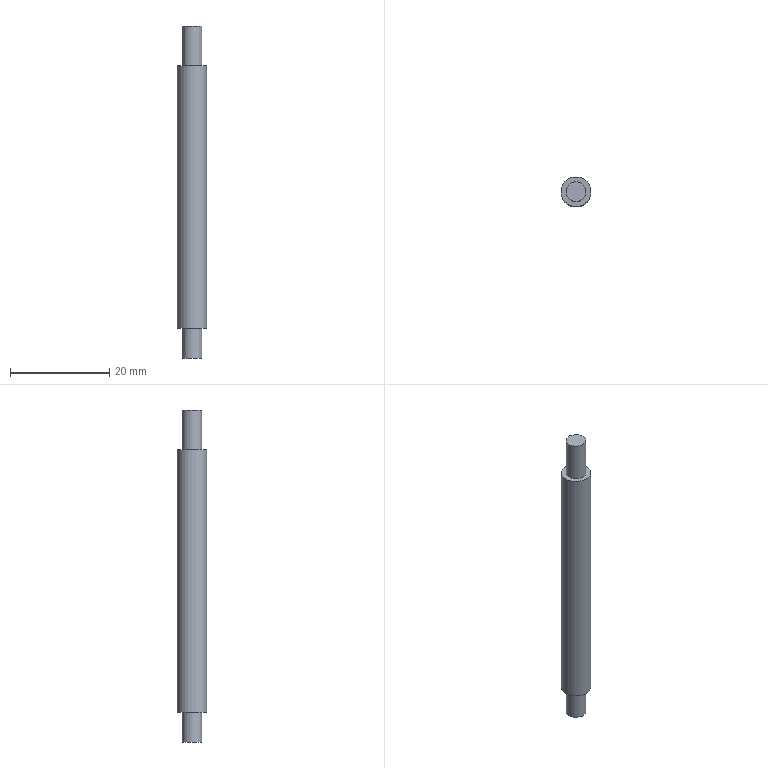Component | NX | CONN_ROD | 1 solid | 7 faces | box 6 x 6 x 67 mm | volume 1674 mm3 | plane 4 | cylinder 3 | commonest cylinder face diameters 4 x2 6 x1
STEP:
#1=CARTESIAN_POINT('',(0.,0.,0.));
#2=DIRECTION('',(0.,0.,1.));
#3=DIRECTION('',(1.,0.,0.));
#4=AXIS2_PLACEMENT_3D('',#1,#2,#3);
#5=CARTESIAN_POINT('',(2.,-10.,96.121));
#6=VERTEX_POINT('',#5);
#7=CARTESIAN_POINT('',(-0.,-10.,96.121));
#8=DIRECTION('',(0.,0.,1.));
#9=DIRECTION('',(1.,0.,0.));
#10=AXIS2_PLACEMENT_3D('',#7,#8,#9);
#11=CIRCLE('',#10,2.);
#12=CARTESIAN_POINT('',(-0.,-10.,96.121));
#13=DIRECTION('',(0.,0.,-1.));
#14=DIRECTION('',(-1.,0.,0.));
#15=AXIS2_PLACEMENT_3D('',#12,#13,#14);
#16=PLANE('',#15);
#17=CARTESIAN_POINT('',(-2.,0.));
#18=CARTESIAN_POINT('',(-2.,3.464));
#19=CARTESIAN_POINT('',(1.,1.732));
#20=CARTESIAN_POINT('',(4.,0.));
#21=CARTESIAN_POINT('',(1.,-1.732));
#22=CARTESIAN_POINT('',(-2.,-3.464));
#23=CARTESIAN_POINT('',(-2.,0.));
#24=(BOUNDED_CURVE()B_SPLINE_CURVE(2,(#17,#18,#19,#20,#21,#22,#23),.UNSPECIFIED.,.T.,.F.)B_SPLINE_CURVE_WITH_KNOTS((1,2,2,2,2,1),(-2.094,0.,2.094,4.189,6.283,8.378),.UNSPECIFIED.)CURVE()GEOMETRIC_REPRESENTATION_ITEM()RATIONAL_B_SPLINE_CURVE((1.,0.5,1.,0.5,1.,0.5,1.))REPRESENTATION_ITEM(''));
#25=(GEOMETRIC_REPRESENTATION_CONTEXT(2)PARAMETRIC_REPRESENTATION_CONTEXT()REPRESENTATION_CONTEXT('',''));
#26=DEFINITIONAL_REPRESENTATION('',(#24),#25);
#27=PCURVE('',#16,#26);
#28=CARTESIAN_POINT('',(-0.,-10.,96.121));
#29=DIRECTION('',(0.,0.,1.));
#30=DIRECTION('',(1.,0.,0.));
#31=AXIS2_PLACEMENT_3D('',#28,#29,#30);
#32=CYLINDRICAL_SURFACE('',#31,2.);
#33=CARTESIAN_POINT('',(0.,0.));
#34=DIRECTION('',(1.,0.));
#35=VECTOR('',#34,1.);
#36=LINE('',#33,#35);
#37=(GEOMETRIC_REPRESENTATION_CONTEXT(2)PARAMETRIC_REPRESENTATION_CONTEXT()REPRESENTATION_CONTEXT('',''));
#38=DEFINITIONAL_REPRESENTATION('',(#36),#37);
#39=PCURVE('',#32,#38);
#40=SURFACE_CURVE('',#11,(#27,#39),.PCURVE_S1.);
#41=EDGE_CURVE('',#6,#6,#40,.T.);
#42=ORIENTED_EDGE('',*,*,#41,.F.);
#43=EDGE_LOOP('',(#42));
#44=FACE_BOUND('',#43,.T.);
#45=ADVANCED_FACE('',(#44),#16,.T.);
#46=CARTESIAN_POINT('',(2.,-10.,102.121));
#47=VERTEX_POINT('',#46);
#48=CARTESIAN_POINT('',(-0.,-10.,102.121));
#49=DIRECTION('',(0.,0.,-1.));
#50=DIRECTION('',(1.,0.,0.));
#51=AXIS2_PLACEMENT_3D('',#48,#49,#50);
#52=CIRCLE('',#51,2.);
#53=CARTESIAN_POINT('',(6.283,6.));
#54=DIRECTION('',(-1.,0.));
#55=VECTOR('',#54,1.);
#56=LINE('',#53,#55);
#57=(GEOMETRIC_REPRESENTATION_CONTEXT(2)PARAMETRIC_REPRESENTATION_CONTEXT()REPRESENTATION_CONTEXT('',''));
#58=DEFINITIONAL_REPRESENTATION('',(#56),#57);
#59=PCURVE('',#32,#58);
#60=CARTESIAN_POINT('',(-0.,-10.,102.121));
#61=DIRECTION('',(0.,0.,-1.));
#62=DIRECTION('',(-1.,0.,0.));
#63=AXIS2_PLACEMENT_3D('',#60,#61,#62);
#64=PLANE('',#63);
#65=CARTESIAN_POINT('',(0.,0.));
#66=DIRECTION('',(-1.,0.));
#67=AXIS2_PLACEMENT_2D('',#65,#66);
#68=CIRCLE('',#67,2.);
#69=(GEOMETRIC_REPRESENTATION_CONTEXT(2)PARAMETRIC_REPRESENTATION_CONTEXT()REPRESENTATION_CONTEXT('',''));
#70=DEFINITIONAL_REPRESENTATION('',(#68),#69);
#71=PCURVE('',#64,#70);
#72=SURFACE_CURVE('',#52,(#59,#71),.PCURVE_S1.);
#73=EDGE_CURVE('',#47,#47,#72,.T.);
#74=ORIENTED_EDGE('',*,*,#73,.T.);
#75=CARTESIAN_POINT('',(2.,-10.,96.121));
#76=CARTESIAN_POINT('',(2.,-10.,102.121));
#77=B_SPLINE_CURVE_WITH_KNOTS('',1,(#75,#76),.UNSPECIFIED.,.F.,.F.,(2,2),(0.,6.),.PIECEWISE_BEZIER_KNOTS.);
#78=CARTESIAN_POINT('',(0.,0.));
#79=DIRECTION('',(0.,1.));
#80=VECTOR('',#79,1.);
#81=LINE('',#78,#80);
#82=(GEOMETRIC_REPRESENTATION_CONTEXT(2)PARAMETRIC_REPRESENTATION_CONTEXT()REPRESENTATION_CONTEXT('',''));
#83=DEFINITIONAL_REPRESENTATION('',(#81),#82);
#84=PCURVE('',#32,#83);
#85=CARTESIAN_POINT('',(6.283,0.));
#86=DIRECTION('',(0.,1.));
#87=VECTOR('',#86,1.);
#88=LINE('',#85,#87);
#89=(GEOMETRIC_REPRESENTATION_CONTEXT(2)PARAMETRIC_REPRESENTATION_CONTEXT()REPRESENTATION_CONTEXT('',''));
#90=DEFINITIONAL_REPRESENTATION('',(#88),#89);
#91=PCURVE('',#32,#90);
#92=SEAM_CURVE('',#77,(#84,#91),.PCURVE_S1.);
#93=EDGE_CURVE('',#6,#47,#92,.T.);
#94=ORIENTED_EDGE('',*,*,#93,.F.);
#95=ORIENTED_EDGE('',*,*,#41,.T.);
#96=ORIENTED_EDGE('',*,*,#93,.T.);
#97=EDGE_LOOP('',(#74,#94,#95,#96));
#98=FACE_BOUND('',#97,.T.);
#99=ADVANCED_FACE('',(#98),#32,.T.);
#100=CARTESIAN_POINT('',(2.,-10.,155.121));
#101=VERTEX_POINT('',#100);
#102=CARTESIAN_POINT('',(-0.,-10.,155.121));
#103=DIRECTION('',(0.,0.,1.));
#104=DIRECTION('',(1.,0.,0.));
#105=AXIS2_PLACEMENT_3D('',#102,#103,#104);
#106=CIRCLE('',#105,2.);
#107=CARTESIAN_POINT('',(-0.,-10.,155.121));
#108=DIRECTION('',(0.,0.,1.));
#109=DIRECTION('',(1.,0.,0.));
#110=AXIS2_PLACEMENT_3D('',#107,#108,#109);
#111=PLANE('',#110);
#112=CARTESIAN_POINT('',(0.,0.));
#113=DIRECTION('',(1.,0.));
#114=AXIS2_PLACEMENT_2D('',#112,#113);
#115=CIRCLE('',#114,2.);
#116=(GEOMETRIC_REPRESENTATION_CONTEXT(2)PARAMETRIC_REPRESENTATION_CONTEXT()REPRESENTATION_CONTEXT('',''));
#117=DEFINITIONAL_REPRESENTATION('',(#115),#116);
#118=PCURVE('',#111,#117);
#119=CARTESIAN_POINT('',(-0.,-10.,155.121));
#120=DIRECTION('',(0.,0.,1.));
#121=DIRECTION('',(1.,0.,0.));
#122=AXIS2_PLACEMENT_3D('',#119,#120,#121);
#123=CYLINDRICAL_SURFACE('',#122,2.);
#124=CARTESIAN_POINT('',(0.,0.));
#125=DIRECTION('',(1.,0.));
#126=VECTOR('',#125,1.);
#127=LINE('',#124,#126);
#128=(GEOMETRIC_REPRESENTATION_CONTEXT(2)PARAMETRIC_REPRESENTATION_CONTEXT()REPRESENTATION_CONTEXT('',''));
#129=DEFINITIONAL_REPRESENTATION('',(#127),#128);
#130=PCURVE('',#123,#129);
#131=SURFACE_CURVE('',#106,(#118,#130),.PCURVE_S1.);
#132=EDGE_CURVE('',#101,#101,#131,.T.);
#133=ORIENTED_EDGE('',*,*,#132,.F.);
#134=EDGE_LOOP('',(#133));
#135=FACE_BOUND('',#134,.T.);
#136=CARTESIAN_POINT('',(3.,-10.,155.121));
#137=VERTEX_POINT('',#136);
#138=CARTESIAN_POINT('',(-0.,-10.,155.121));
#139=DIRECTION('',(0.,0.,1.));
#140=DIRECTION('',(1.,0.,0.));
#141=AXIS2_PLACEMENT_3D('',#138,#139,#140);
#142=CIRCLE('',#141,3.);
#143=CARTESIAN_POINT('',(0.,0.));
#144=DIRECTION('',(1.,0.));
#145=AXIS2_PLACEMENT_2D('',#143,#144);
#146=CIRCLE('',#145,3.);
#147=(GEOMETRIC_REPRESENTATION_CONTEXT(2)PARAMETRIC_REPRESENTATION_CONTEXT()REPRESENTATION_CONTEXT('',''));
#148=DEFINITIONAL_REPRESENTATION('',(#146),#147);
#149=PCURVE('',#111,#148);
#150=CARTESIAN_POINT('',(-0.,-10.,102.121));
#151=DIRECTION('',(0.,0.,1.));
#152=DIRECTION('',(1.,0.,0.));
#153=AXIS2_PLACEMENT_3D('',#150,#151,#152);
#154=CYLINDRICAL_SURFACE('',#153,3.);
#155=CARTESIAN_POINT('',(0.,53.));
#156=DIRECTION('',(1.,0.));
#157=VECTOR('',#156,1.);
#158=LINE('',#155,#157);
#159=(GEOMETRIC_REPRESENTATION_CONTEXT(2)PARAMETRIC_REPRESENTATION_CONTEXT()REPRESENTATION_CONTEXT('',''));
#160=DEFINITIONAL_REPRESENTATION('',(#158),#159);
#161=PCURVE('',#154,#160);
#162=SURFACE_CURVE('',#142,(#149,#161),.PCURVE_S1.);
#163=EDGE_CURVE('',#137,#137,#162,.T.);
#164=ORIENTED_EDGE('',*,*,#163,.T.);
#165=EDGE_LOOP('',(#164));
#166=FACE_BOUND('',#165,.T.);
#167=ADVANCED_FACE('',(#135,#166),#111,.T.);
#168=ORIENTED_EDGE('',*,*,#73,.F.);
#169=EDGE_LOOP('',(#168));
#170=FACE_BOUND('',#169,.T.);
#171=CARTESIAN_POINT('',(3.,-10.,102.121));
#172=VERTEX_POINT('',#171);
#173=CARTESIAN_POINT('',(-0.,-10.,102.121));
#174=DIRECTION('',(0.,0.,1.));
#175=DIRECTION('',(1.,0.,0.));
#176=AXIS2_PLACEMENT_3D('',#173,#174,#175);
#177=CIRCLE('',#176,3.);
#178=CARTESIAN_POINT('',(-3.,0.));
#179=CARTESIAN_POINT('',(-3.,5.196));
#180=CARTESIAN_POINT('',(1.5,2.598));
#181=CARTESIAN_POINT('',(6.,0.));
#182=CARTESIAN_POINT('',(1.5,-2.598));
#183=CARTESIAN_POINT('',(-3.,-5.196));
#184=CARTESIAN_POINT('',(-3.,0.));
#185=(BOUNDED_CURVE()B_SPLINE_CURVE(2,(#178,#179,#180,#181,#182,#183,#184),.UNSPECIFIED.,.T.,.F.)B_SPLINE_CURVE_WITH_KNOTS((1,2,2,2,2,1),(-2.094,0.,2.094,4.189,6.283,8.378),.UNSPECIFIED.)CURVE()GEOMETRIC_REPRESENTATION_ITEM()RATIONAL_B_SPLINE_CURVE((1.,0.5,1.,0.5,1.,0.5,1.))REPRESENTATION_ITEM(''));
#186=(GEOMETRIC_REPRESENTATION_CONTEXT(2)PARAMETRIC_REPRESENTATION_CONTEXT()REPRESENTATION_CONTEXT('',''));
#187=DEFINITIONAL_REPRESENTATION('',(#185),#186);
#188=PCURVE('',#64,#187);
#189=CARTESIAN_POINT('',(0.,0.));
#190=DIRECTION('',(1.,0.));
#191=VECTOR('',#190,1.);
#192=LINE('',#189,#191);
#193=(GEOMETRIC_REPRESENTATION_CONTEXT(2)PARAMETRIC_REPRESENTATION_CONTEXT()REPRESENTATION_CONTEXT('',''));
#194=DEFINITIONAL_REPRESENTATION('',(#192),#193);
#195=PCURVE('',#154,#194);
#196=SURFACE_CURVE('',#177,(#188,#195),.PCURVE_S1.);
#197=EDGE_CURVE('',#172,#172,#196,.T.);
#198=ORIENTED_EDGE('',*,*,#197,.F.);
#199=EDGE_LOOP('',(#198));
#200=FACE_BOUND('',#199,.T.);
#201=ADVANCED_FACE('',(#170,#200),#64,.T.);
#202=ORIENTED_EDGE('',*,*,#163,.F.);
#203=CARTESIAN_POINT('',(3.,-10.,102.121));
#204=CARTESIAN_POINT('',(3.,-10.,155.121));
#205=B_SPLINE_CURVE_WITH_KNOTS('',1,(#203,#204),.UNSPECIFIED.,.F.,.F.,(2,2),(0.,53.),.PIECEWISE_BEZIER_KNOTS.);
#206=CARTESIAN_POINT('',(0.,0.));
#207=DIRECTION('',(0.,1.));
#208=VECTOR('',#207,1.);
#209=LINE('',#206,#208);
#210=(GEOMETRIC_REPRESENTATION_CONTEXT(2)PARAMETRIC_REPRESENTATION_CONTEXT()REPRESENTATION_CONTEXT('',''));
#211=DEFINITIONAL_REPRESENTATION('',(#209),#210);
#212=PCURVE('',#154,#211);
#213=CARTESIAN_POINT('',(6.283,0.));
#214=DIRECTION('',(0.,1.));
#215=VECTOR('',#214,1.);
#216=LINE('',#213,#215);
#217=(GEOMETRIC_REPRESENTATION_CONTEXT(2)PARAMETRIC_REPRESENTATION_CONTEXT()REPRESENTATION_CONTEXT('',''));
#218=DEFINITIONAL_REPRESENTATION('',(#216),#217);
#219=PCURVE('',#154,#218);
#220=SEAM_CURVE('',#205,(#212,#219),.PCURVE_S1.);
#221=EDGE_CURVE('',#172,#137,#220,.T.);
#222=ORIENTED_EDGE('',*,*,#221,.F.);
#223=ORIENTED_EDGE('',*,*,#197,.T.);
#224=ORIENTED_EDGE('',*,*,#221,.T.);
#225=EDGE_LOOP('',(#202,#222,#223,#224));
#226=FACE_BOUND('',#225,.T.);
#227=ADVANCED_FACE('',(#226),#154,.T.);
#228=CARTESIAN_POINT('',(2.,-10.,163.121));
#229=VERTEX_POINT('',#228);
#230=CARTESIAN_POINT('',(-0.,-10.,163.121));
#231=DIRECTION('',(0.,0.,1.));
#232=DIRECTION('',(1.,0.,0.));
#233=AXIS2_PLACEMENT_3D('',#230,#231,#232);
#234=CIRCLE('',#233,2.);
#235=CARTESIAN_POINT('',(-0.,-10.,163.121));
#236=DIRECTION('',(0.,0.,1.));
#237=DIRECTION('',(1.,0.,0.));
#238=AXIS2_PLACEMENT_3D('',#235,#236,#237);
#239=PLANE('',#238);
#240=CARTESIAN_POINT('',(0.,0.));
#241=DIRECTION('',(1.,0.));
#242=AXIS2_PLACEMENT_2D('',#240,#241);
#243=CIRCLE('',#242,2.);
#244=(GEOMETRIC_REPRESENTATION_CONTEXT(2)PARAMETRIC_REPRESENTATION_CONTEXT()REPRESENTATION_CONTEXT('',''));
#245=DEFINITIONAL_REPRESENTATION('',(#243),#244);
#246=PCURVE('',#239,#245);
#247=CARTESIAN_POINT('',(0.,8.));
#248=DIRECTION('',(1.,0.));
#249=VECTOR('',#248,1.);
#250=LINE('',#247,#249);
#251=(GEOMETRIC_REPRESENTATION_CONTEXT(2)PARAMETRIC_REPRESENTATION_CONTEXT()REPRESENTATION_CONTEXT('',''));
#252=DEFINITIONAL_REPRESENTATION('',(#250),#251);
#253=PCURVE('',#123,#252);
#254=SURFACE_CURVE('',#234,(#246,#253),.PCURVE_S1.);
#255=EDGE_CURVE('',#229,#229,#254,.T.);
#256=ORIENTED_EDGE('',*,*,#255,.T.);
#257=EDGE_LOOP('',(#256));
#258=FACE_BOUND('',#257,.T.);
#259=ADVANCED_FACE('',(#258),#239,.T.);
#260=ORIENTED_EDGE('',*,*,#255,.F.);
#261=CARTESIAN_POINT('',(2.,-10.,155.121));
#262=CARTESIAN_POINT('',(2.,-10.,163.121));
#263=B_SPLINE_CURVE_WITH_KNOTS('',1,(#261,#262),.UNSPECIFIED.,.F.,.F.,(2,2),(0.,8.),.PIECEWISE_BEZIER_KNOTS.);
#264=CARTESIAN_POINT('',(0.,0.));
#265=DIRECTION('',(0.,1.));
#266=VECTOR('',#265,1.);
#267=LINE('',#264,#266);
#268=(GEOMETRIC_REPRESENTATION_CONTEXT(2)PARAMETRIC_REPRESENTATION_CONTEXT()REPRESENTATION_CONTEXT('',''));
#269=DEFINITIONAL_REPRESENTATION('',(#267),#268);
#270=PCURVE('',#123,#269);
#271=CARTESIAN_POINT('',(6.283,0.));
#272=DIRECTION('',(0.,1.));
#273=VECTOR('',#272,1.);
#274=LINE('',#271,#273);
#275=(GEOMETRIC_REPRESENTATION_CONTEXT(2)PARAMETRIC_REPRESENTATION_CONTEXT()REPRESENTATION_CONTEXT('',''));
#276=DEFINITIONAL_REPRESENTATION('',(#274),#275);
#277=PCURVE('',#123,#276);
#278=SEAM_CURVE('',#263,(#270,#277),.PCURVE_S1.);
#279=EDGE_CURVE('',#101,#229,#278,.T.);
#280=ORIENTED_EDGE('',*,*,#279,.F.);
#281=ORIENTED_EDGE('',*,*,#132,.T.);
#282=ORIENTED_EDGE('',*,*,#279,.T.);
#283=EDGE_LOOP('',(#260,#280,#281,#282));
#284=FACE_BOUND('',#283,.T.);
#285=ADVANCED_FACE('',(#284),#123,.T.);
#286=CLOSED_SHELL('',(#45,#99,#167,#201,#227,#259,#285));
#287=MANIFOLD_SOLID_BREP('',#286);
#288=(LENGTH_UNIT()NAMED_UNIT(*)SI_UNIT(.MILLI.,.METRE.));
#289=UNCERTAINTY_MEASURE_WITH_UNIT(LENGTH_MEASURE(0.00001),#288,'','');
#290=(NAMED_UNIT(*)PLANE_ANGLE_UNIT()SI_UNIT($,.RADIAN.));
#291=(NAMED_UNIT(*)SI_UNIT($,.STERADIAN.)SOLID_ANGLE_UNIT());
#292=(GEOMETRIC_REPRESENTATION_CONTEXT(3)GLOBAL_UNCERTAINTY_ASSIGNED_CONTEXT((#289))GLOBAL_UNIT_ASSIGNED_CONTEXT((#288,#290,#291))REPRESENTATION_CONTEXT('',''));
#293=ADVANCED_BREP_SHAPE_REPRESENTATION('',(#4,#287),#292);